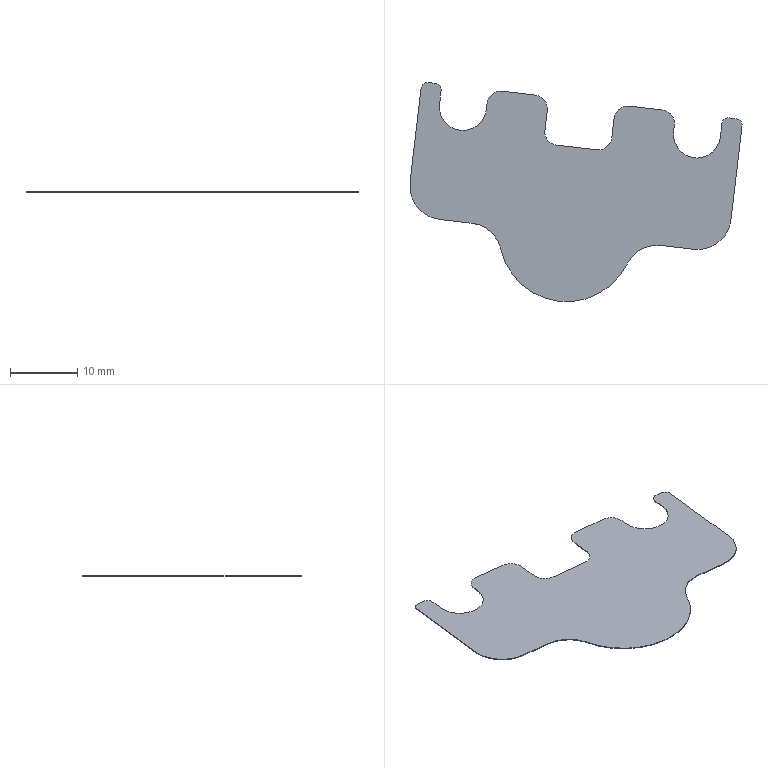Component | SolidWorks | 8TC-A17001-90-07AdjustmentShim-1 | 1 solid | 34 faces | box 49.35 x 32.55 x 0.1 mm | volume 96 mm3 | cylinder 17 | plane 17 | commonest cylinder face diameters 4 x6 10 x4 2 x4 7 x2 20 x1 | material SUS304
build123d program:
from build123d import *

# Parameters (mm, degrees)
BOSS_EXTRUDE1_DEPTH = 0.1
FILLET_R5_R         = 5
FILLET2_R           = 1
FILLET3_R           = 2


with BuildPart() as part:
    # Sketch1 → Boss-Extrude1 (new body)
    with BuildSketch(Plane.XY):
        with BuildLine():
            Line((21, 17), (21, 20))
            Line((21, 20), (24, 20))
            Line((24, 20), (24, 0))
            Line((24, 0), (10, 0))
            ThreePointArc((10, 0), (0, -10), (-10, 0))
            Line((-10, 0), (-24, 0))
            Line((-24, 0), (-24, 20))
            Line((-24, 20), (-21, 20))
            Line((-21, 20), (-21, 17))
            ThreePointArc((-21, 17), (-17.5, 13.5), (-14, 17))
            Line((-14, 17), (-14, 20))
            Line((-14, 20), (-5, 20))
            Line((-5, 20), (-5, 13))
            Line((-5, 13), (5, 13))
            Line((5, 13), (5, 20))
            Line((5, 20), (14, 20))
            Line((14, 20), (14, 17))
            ThreePointArc((14, 17), (17.5, 13.5), (21, 17))
        make_face()
    extrude(amount=BOSS_EXTRUDE1_DEPTH)

    # Fillet R5
    fillet_r5_edges = [part.edges().sort_by_distance(p)[0] for p in [
        (24, 0, 0.05),
        (10, 0, 0.05),
        (-10, 0, 0.05),
        (-24, 0, 0.05),
    ]]
    fillet(fillet_r5_edges, radius=FILLET_R5_R)

    # Fillet2
    fillet2_edges = [part.edges().sort_by_distance(p)[0] for p in [
        (21, 20, 0.05),
        (24, 20, 0.05),
        (-24, 20, 0.05),
        (-21, 20, 0.05),
    ]]
    fillet(fillet2_edges, radius=FILLET2_R)

    # Fillet3
    fillet3_edges = [part.edges().sort_by_distance(p)[0] for p in [
        (-14, 20, 0.05),
        (-5, 20, 0.05),
        (-5, 13, 0.05),
        (5, 13, 0.05),
        (5, 20, 0.05),
        (14, 20, 0.05),
    ]]
    fillet(fillet3_edges, radius=FILLET3_R)


solid = part.part

# Placed as in the assembly
solid = solid.moved(Location((-2.188, -110.884, -136.2), (0, 0, -6.7)))